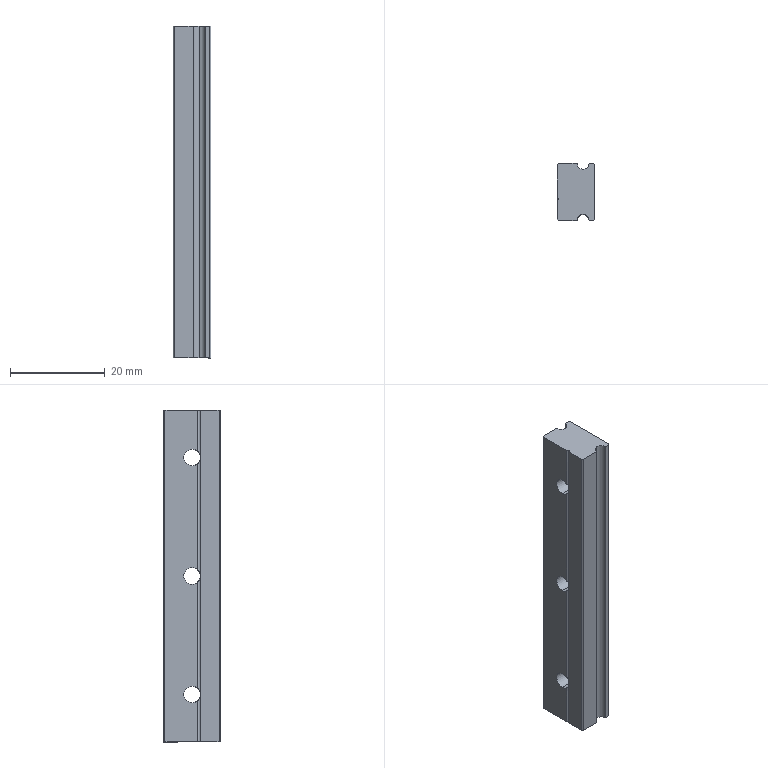Component | SolidWorks | 1-VASP2004MANIFOLD_SOLID_BREP_99-01-2 | 1 solid | 32 faces | volume 5872 mm3 | cylinder 16 | plane 16 | commonest cylinder face diameters 6 x6 3.5 x6 2.5 x3 0.6 x1